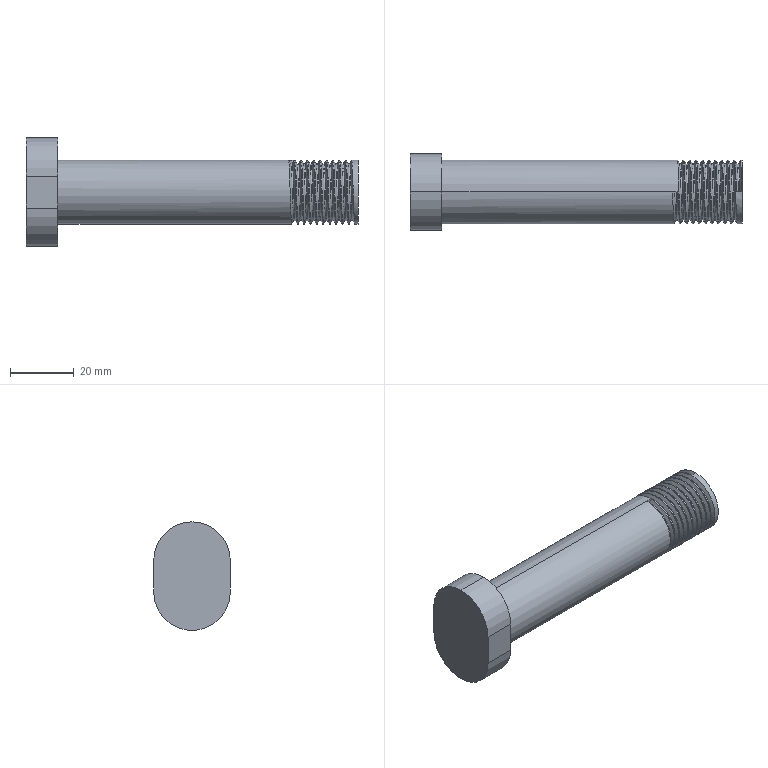Component | SolidWorks | pengunci-3 | 1 solid | 35 faces | volume 35725 mm3 | cylinder 25 | plane 7 | spline 3 | commonest cylinder face diameters 20 x22 24 x3